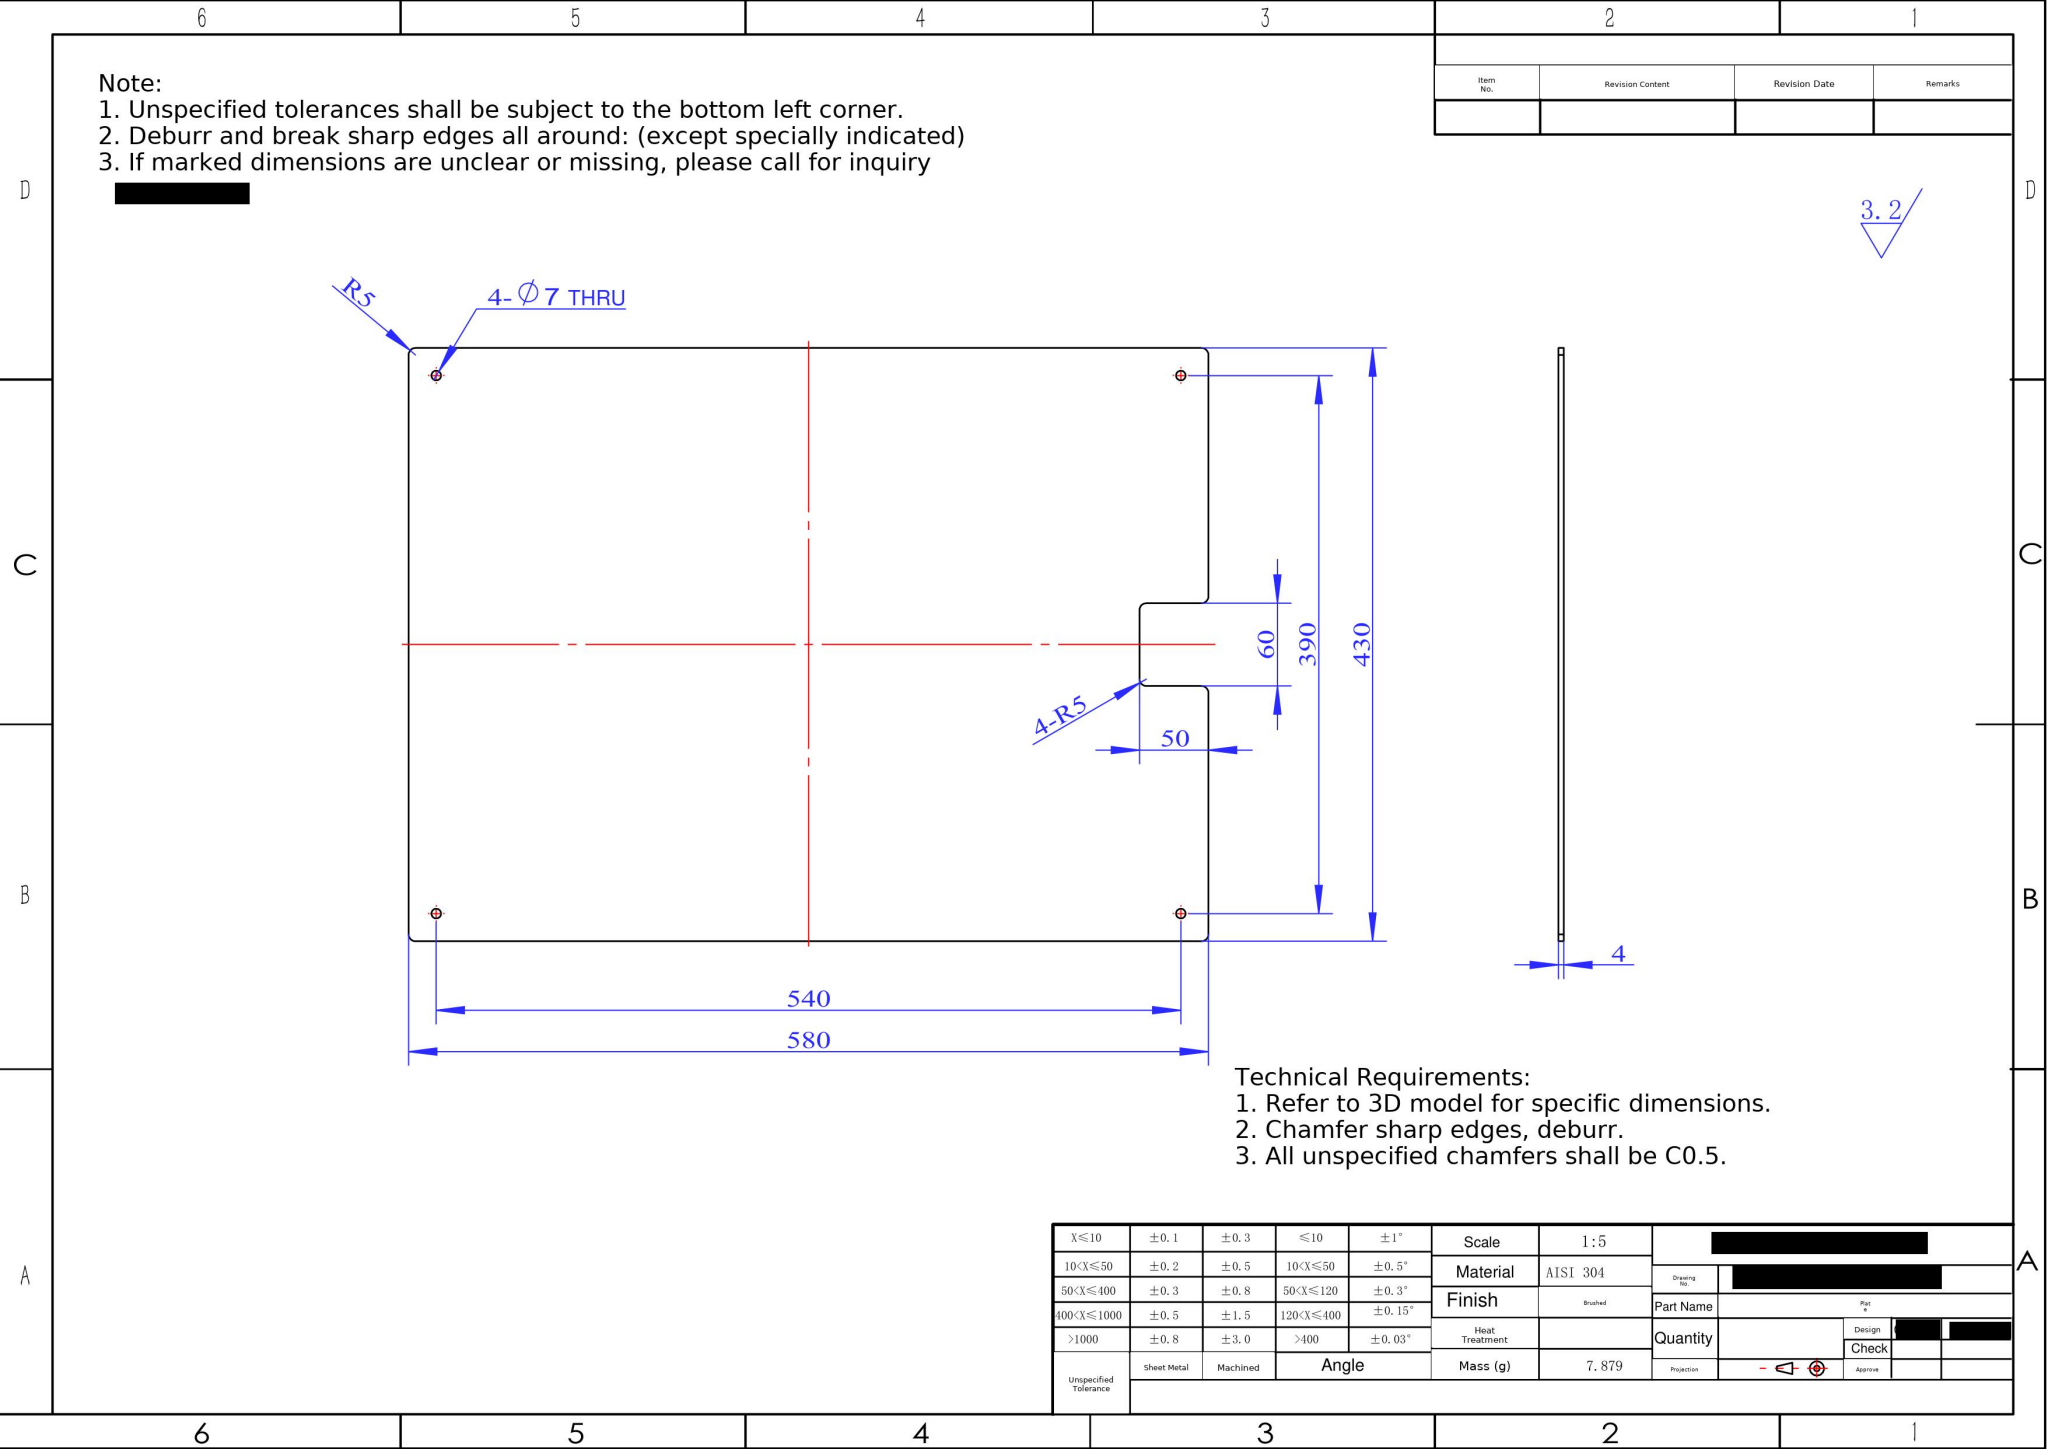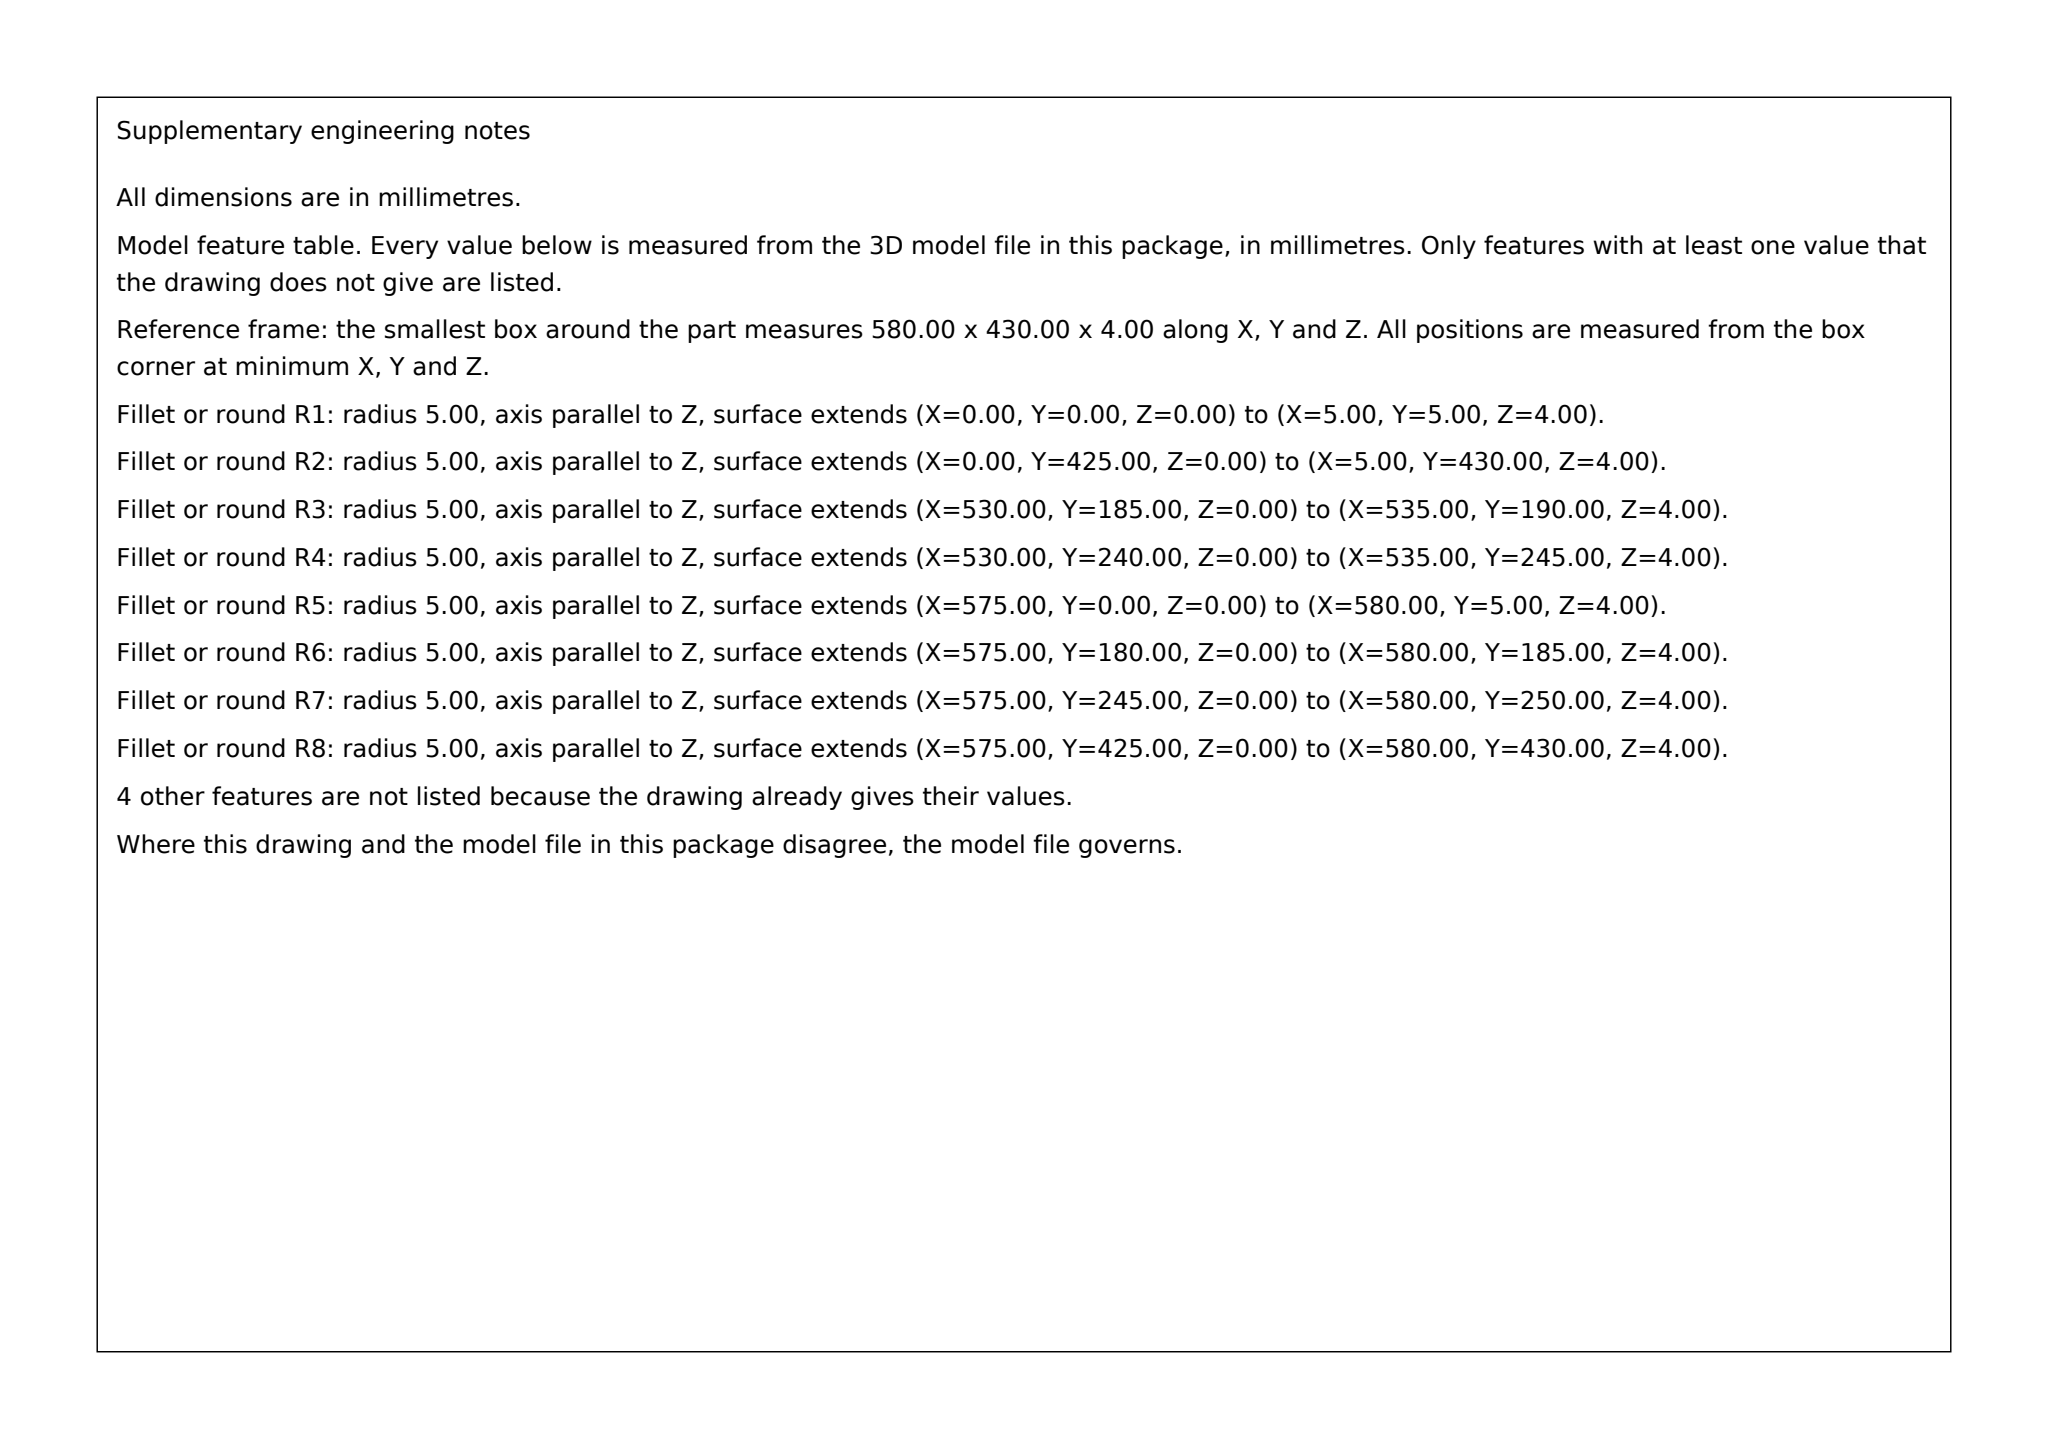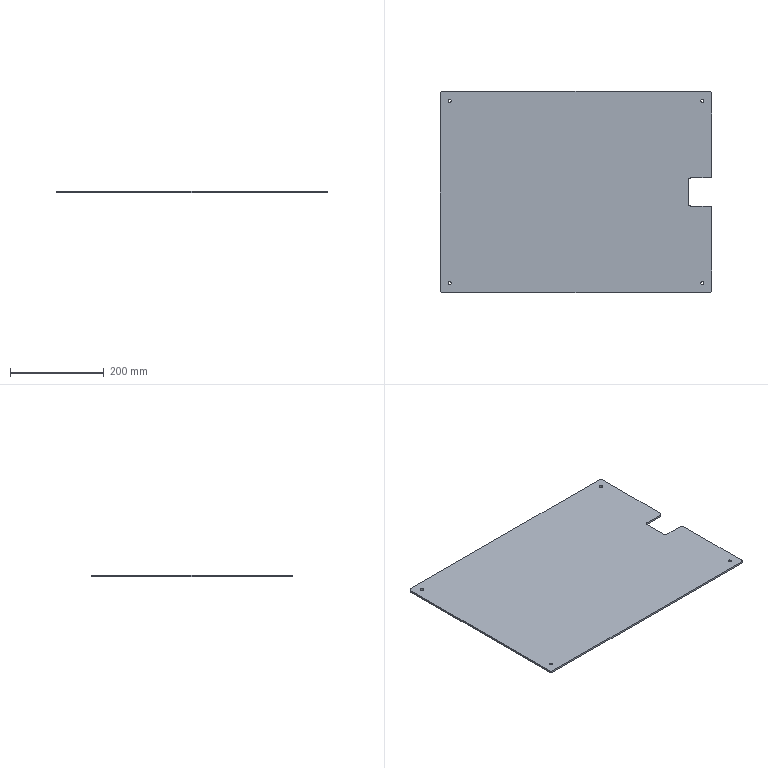Part | SolidWorks | mm | material AISI 304 | 1 solid | 26 faces | box 580 x 430 x 4 mm | volume 984898 mm3 | cylinder 16 | plane 10 | commonest cylinder face diameters 7 x8 10 x8
build123d program:
from build123d import *

# Parameters (mm, degrees)
SKETCH1_W           = 580
SKETCH1_H           = 430
BOSS_EXTRUDE1_DEPTH = 4
FILLET1_R           = 5
SKETCH2_W           = 50
SKETCH2_H           = 60
CUT_EXTRUDE1_DEPTH  = 723.022
FILLET2_R           = 5
SKETCH3_R           = 3.5
CUT_EXTRUDE2_DEPTH  = 723.022


with BuildPart() as part:
    # Sketch1 → Boss-Extrude1 (new body)
    with BuildSketch(Plane.XY):
        with Locations((290, -215)):
            Rectangle(SKETCH1_W, SKETCH1_H)
    extrude(amount=BOSS_EXTRUDE1_DEPTH)

    # Fillet1
    fillet1_edges = [part.edges().sort_by_distance(p)[0] for p in [
        (580, -430, 2),
        (0, -430, 2),
        (0, 0, 2),
        (580, 0, 2),
    ]]
    fillet(fillet1_edges, radius=FILLET1_R)

    # Sketch2 → Cut-Extrude1 (cut, through all)
    with BuildSketch(Plane(origin=(0, 0, 0), x_dir=(-1, 0, 0), z_dir=(0, 0, -1))):
        with Locations((-555, -215)):
            Rectangle(SKETCH2_W, SKETCH2_H)
    extrude(amount=-CUT_EXTRUDE1_DEPTH, mode=Mode.SUBTRACT)

    # Fillet2
    fillet2_edges = [part.edges().sort_by_distance(p)[0] for p in [
        (580, -245, 2),
        (580, -185, 2),
        (530, -185, 2),
        (530, -245, 2),
    ]]
    fillet(fillet2_edges, radius=FILLET2_R)

    # Sketch3 → Cut-Extrude2 (cut, through all)
    with BuildSketch(Plane(origin=(0, 0, 0), x_dir=(-1, 0, 0), z_dir=(0, 0, -1))):
        with Locations((-560, -20)):
            Circle(SKETCH3_R)
        with Locations((-560, -410)):
            Circle(SKETCH3_R)
        with Locations((-20, -20)):
            Circle(SKETCH3_R)
        with Locations((-20, -410)):
            Circle(SKETCH3_R)
    extrude(amount=-CUT_EXTRUDE2_DEPTH, mode=Mode.SUBTRACT)


solid = part.part
STEP:
#1=CARTESIAN_POINT('',(563.5,-410.,4.));
#2=VERTEX_POINT('',#1);
#3=CARTESIAN_POINT('',(556.5,-410.,4.));
#4=VERTEX_POINT('',#3);
#5=CARTESIAN_POINT('',(560.,-410.,4.));
#6=DIRECTION('',(0.,0.,-1.));
#7=DIRECTION('',(-1.,0.,0.));
#8=AXIS2_PLACEMENT_3D('',#5,#6,#7);
#9=CIRCLE('',#8,3.5);
#10=EDGE_CURVE('',#2,#4,#9,.T.);
#11=ORIENTED_EDGE('',*,*,#10,.F.);
#12=CARTESIAN_POINT('',(563.5,-410.,0.));
#13=VERTEX_POINT('',#12);
#14=CARTESIAN_POINT('',(563.5,-410.,4.));
#15=DIRECTION('',(0.,0.,-1.));
#16=VECTOR('',#15,1000.);
#17=LINE('',#14,#16);
#18=EDGE_CURVE('',#2,#13,#17,.T.);
#19=ORIENTED_EDGE('',*,*,#18,.T.);
#20=CARTESIAN_POINT('',(556.5,-410.,0.));
#21=VERTEX_POINT('',#20);
#22=CARTESIAN_POINT('',(560.,-410.,0.));
#23=DIRECTION('',(0.,0.,-1.));
#24=DIRECTION('',(-1.,0.,0.));
#25=AXIS2_PLACEMENT_3D('',#22,#23,#24);
#26=CIRCLE('',#25,3.5);
#27=EDGE_CURVE('',#13,#21,#26,.T.);
#28=ORIENTED_EDGE('',*,*,#27,.T.);
#29=CARTESIAN_POINT('',(556.5,-410.,4.));
#30=DIRECTION('',(0.,0.,-1.));
#31=VECTOR('',#30,1000.);
#32=LINE('',#29,#31);
#33=EDGE_CURVE('',#4,#21,#32,.T.);
#34=ORIENTED_EDGE('',*,*,#33,.F.);
#35=EDGE_LOOP('',(#11,#19,#28,#34));
#36=FACE_OUTER_BOUND('',#35,.T.);
#37=CARTESIAN_POINT('',(560.,-410.,4.));
#38=DIRECTION('',(0.,0.,-1.));
#39=DIRECTION('',(-1.,0.,0.));
#40=AXIS2_PLACEMENT_3D('',#37,#38,#39);
#41=CYLINDRICAL_SURFACE('',#40,3.5);
#42=ADVANCED_FACE('',(#36),#41,.F.);
#43=CARTESIAN_POINT('',(23.5,-20.,4.));
#44=VERTEX_POINT('',#43);
#45=CARTESIAN_POINT('',(16.5,-20.,4.));
#46=VERTEX_POINT('',#45);
#47=CARTESIAN_POINT('',(20.,-20.,4.));
#48=DIRECTION('',(0.,0.,-1.));
#49=DIRECTION('',(-1.,0.,0.));
#50=AXIS2_PLACEMENT_3D('',#47,#48,#49);
#51=CIRCLE('',#50,3.5);
#52=EDGE_CURVE('',#44,#46,#51,.T.);
#53=ORIENTED_EDGE('',*,*,#52,.F.);
#54=CARTESIAN_POINT('',(23.5,-20.,0.));
#55=VERTEX_POINT('',#54);
#56=CARTESIAN_POINT('',(23.5,-20.,4.));
#57=DIRECTION('',(0.,0.,-1.));
#58=VECTOR('',#57,1000.);
#59=LINE('',#56,#58);
#60=EDGE_CURVE('',#44,#55,#59,.T.);
#61=ORIENTED_EDGE('',*,*,#60,.T.);
#62=CARTESIAN_POINT('',(16.5,-20.,0.));
#63=VERTEX_POINT('',#62);
#64=CARTESIAN_POINT('',(20.,-20.,0.));
#65=DIRECTION('',(0.,0.,-1.));
#66=DIRECTION('',(-1.,0.,0.));
#67=AXIS2_PLACEMENT_3D('',#64,#65,#66);
#68=CIRCLE('',#67,3.5);
#69=EDGE_CURVE('',#55,#63,#68,.T.);
#70=ORIENTED_EDGE('',*,*,#69,.T.);
#71=CARTESIAN_POINT('',(16.5,-20.,4.));
#72=DIRECTION('',(0.,0.,-1.));
#73=VECTOR('',#72,1000.);
#74=LINE('',#71,#73);
#75=EDGE_CURVE('',#46,#63,#74,.T.);
#76=ORIENTED_EDGE('',*,*,#75,.F.);
#77=EDGE_LOOP('',(#53,#61,#70,#76));
#78=FACE_OUTER_BOUND('',#77,.T.);
#79=CARTESIAN_POINT('',(20.,-20.,4.));
#80=DIRECTION('',(0.,0.,-1.));
#81=DIRECTION('',(-1.,0.,0.));
#82=AXIS2_PLACEMENT_3D('',#79,#80,#81);
#83=CYLINDRICAL_SURFACE('',#82,3.5);
#84=ADVANCED_FACE('',(#78),#83,.F.);
#85=CARTESIAN_POINT('',(23.5,-410.,4.));
#86=VERTEX_POINT('',#85);
#87=CARTESIAN_POINT('',(16.5,-410.,4.));
#88=VERTEX_POINT('',#87);
#89=CARTESIAN_POINT('',(20.,-410.,4.));
#90=DIRECTION('',(0.,0.,-1.));
#91=DIRECTION('',(-1.,0.,0.));
#92=AXIS2_PLACEMENT_3D('',#89,#90,#91);
#93=CIRCLE('',#92,3.5);
#94=EDGE_CURVE('',#86,#88,#93,.T.);
#95=ORIENTED_EDGE('',*,*,#94,.F.);
#96=CARTESIAN_POINT('',(23.5,-410.,0.));
#97=VERTEX_POINT('',#96);
#98=CARTESIAN_POINT('',(23.5,-410.,4.));
#99=DIRECTION('',(0.,0.,-1.));
#100=VECTOR('',#99,1000.);
#101=LINE('',#98,#100);
#102=EDGE_CURVE('',#86,#97,#101,.T.);
#103=ORIENTED_EDGE('',*,*,#102,.T.);
#104=CARTESIAN_POINT('',(16.5,-410.,0.));
#105=VERTEX_POINT('',#104);
#106=CARTESIAN_POINT('',(20.,-410.,0.));
#107=DIRECTION('',(0.,0.,-1.));
#108=DIRECTION('',(-1.,0.,0.));
#109=AXIS2_PLACEMENT_3D('',#106,#107,#108);
#110=CIRCLE('',#109,3.5);
#111=EDGE_CURVE('',#97,#105,#110,.T.);
#112=ORIENTED_EDGE('',*,*,#111,.T.);
#113=CARTESIAN_POINT('',(16.5,-410.,4.));
#114=DIRECTION('',(0.,0.,-1.));
#115=VECTOR('',#114,1000.);
#116=LINE('',#113,#115);
#117=EDGE_CURVE('',#88,#105,#116,.T.);
#118=ORIENTED_EDGE('',*,*,#117,.F.);
#119=EDGE_LOOP('',(#95,#103,#112,#118));
#120=FACE_OUTER_BOUND('',#119,.T.);
#121=CARTESIAN_POINT('',(20.,-410.,4.));
#122=DIRECTION('',(0.,0.,-1.));
#123=DIRECTION('',(-1.,0.,0.));
#124=AXIS2_PLACEMENT_3D('',#121,#122,#123);
#125=CYLINDRICAL_SURFACE('',#124,3.5);
#126=ADVANCED_FACE('',(#120),#125,.F.);
#127=CARTESIAN_POINT('',(563.5,-20.,4.));
#128=VERTEX_POINT('',#127);
#129=CARTESIAN_POINT('',(556.5,-20.,4.));
#130=VERTEX_POINT('',#129);
#131=CARTESIAN_POINT('',(560.,-20.,4.));
#132=DIRECTION('',(0.,0.,-1.));
#133=DIRECTION('',(-1.,0.,0.));
#134=AXIS2_PLACEMENT_3D('',#131,#132,#133);
#135=CIRCLE('',#134,3.5);
#136=EDGE_CURVE('',#128,#130,#135,.T.);
#137=ORIENTED_EDGE('',*,*,#136,.F.);
#138=CARTESIAN_POINT('',(563.5,-20.,0.));
#139=VERTEX_POINT('',#138);
#140=CARTESIAN_POINT('',(563.5,-20.,4.));
#141=DIRECTION('',(0.,0.,-1.));
#142=VECTOR('',#141,1000.);
#143=LINE('',#140,#142);
#144=EDGE_CURVE('',#128,#139,#143,.T.);
#145=ORIENTED_EDGE('',*,*,#144,.T.);
#146=CARTESIAN_POINT('',(556.5,-20.,0.));
#147=VERTEX_POINT('',#146);
#148=CARTESIAN_POINT('',(560.,-20.,0.));
#149=DIRECTION('',(0.,0.,-1.));
#150=DIRECTION('',(-1.,0.,0.));
#151=AXIS2_PLACEMENT_3D('',#148,#149,#150);
#152=CIRCLE('',#151,3.5);
#153=EDGE_CURVE('',#139,#147,#152,.T.);
#154=ORIENTED_EDGE('',*,*,#153,.T.);
#155=CARTESIAN_POINT('',(556.5,-20.,4.));
#156=DIRECTION('',(0.,0.,-1.));
#157=VECTOR('',#156,1000.);
#158=LINE('',#155,#157);
#159=EDGE_CURVE('',#130,#147,#158,.T.);
#160=ORIENTED_EDGE('',*,*,#159,.F.);
#161=EDGE_LOOP('',(#137,#145,#154,#160));
#162=FACE_OUTER_BOUND('',#161,.T.);
#163=CARTESIAN_POINT('',(560.,-20.,4.));
#164=DIRECTION('',(0.,0.,-1.));
#165=DIRECTION('',(-1.,0.,0.));
#166=AXIS2_PLACEMENT_3D('',#163,#164,#165);
#167=CYLINDRICAL_SURFACE('',#166,3.5);
#168=ADVANCED_FACE('',(#162),#167,.F.);
#169=CARTESIAN_POINT('',(580.,-180.,4.));
#170=VERTEX_POINT('',#169);
#171=CARTESIAN_POINT('',(580.,-5.,4.));
#172=VERTEX_POINT('',#171);
#173=CARTESIAN_POINT('',(580.,-430.,4.));
#174=DIRECTION('',(0.,1.,0.));
#175=VECTOR('',#174,1000.);
#176=LINE('',#173,#175);
#177=EDGE_CURVE('',#170,#172,#176,.T.);
#178=ORIENTED_EDGE('',*,*,#177,.F.);
#179=CARTESIAN_POINT('',(580.,-180.,0.));
#180=VERTEX_POINT('',#179);
#181=CARTESIAN_POINT('',(580.,-180.,4.));
#182=DIRECTION('',(0.,0.,-1.));
#183=VECTOR('',#182,1000.);
#184=LINE('',#181,#183);
#185=EDGE_CURVE('',#170,#180,#184,.T.);
#186=ORIENTED_EDGE('',*,*,#185,.T.);
#187=CARTESIAN_POINT('',(580.,-5.,0.));
#188=VERTEX_POINT('',#187);
#189=CARTESIAN_POINT('',(580.,-430.,0.));
#190=DIRECTION('',(0.,1.,0.));
#191=VECTOR('',#190,1000.);
#192=LINE('',#189,#191);
#193=EDGE_CURVE('',#180,#188,#192,.T.);
#194=ORIENTED_EDGE('',*,*,#193,.T.);
#195=CARTESIAN_POINT('',(580.,-5.,4.));
#196=DIRECTION('',(0.,0.,1.));
#197=VECTOR('',#196,1000.);
#198=LINE('',#195,#197);
#199=EDGE_CURVE('',#188,#172,#198,.T.);
#200=ORIENTED_EDGE('',*,*,#199,.T.);
#201=EDGE_LOOP('',(#178,#186,#194,#200));
#202=FACE_OUTER_BOUND('',#201,.T.);
#203=CARTESIAN_POINT('',(580.,-430.,4.));
#204=DIRECTION('',(-1.,0.,0.));
#205=DIRECTION('',(0.,0.,1.));
#206=AXIS2_PLACEMENT_3D('',#203,#204,#205);
#207=PLANE('',#206);
#208=ADVANCED_FACE('',(#202),#207,.F.);
#209=CARTESIAN_POINT('',(580.,-425.,0.));
#210=VERTEX_POINT('',#209);
#211=CARTESIAN_POINT('',(580.,-250.,0.));
#212=VERTEX_POINT('',#211);
#213=CARTESIAN_POINT('',(580.,-430.,0.));
#214=DIRECTION('',(0.,1.,0.));
#215=VECTOR('',#214,1000.);
#216=LINE('',#213,#215);
#217=EDGE_CURVE('',#210,#212,#216,.T.);
#218=ORIENTED_EDGE('',*,*,#217,.T.);
#219=CARTESIAN_POINT('',(580.,-250.,4.));
#220=VERTEX_POINT('',#219);
#221=CARTESIAN_POINT('',(580.,-250.,4.));
#222=DIRECTION('',(0.,0.,1.));
#223=VECTOR('',#222,1000.);
#224=LINE('',#221,#223);
#225=EDGE_CURVE('',#212,#220,#224,.T.);
#226=ORIENTED_EDGE('',*,*,#225,.T.);
#227=CARTESIAN_POINT('',(580.,-425.,4.));
#228=VERTEX_POINT('',#227);
#229=CARTESIAN_POINT('',(580.,-430.,4.));
#230=DIRECTION('',(0.,1.,0.));
#231=VECTOR('',#230,1000.);
#232=LINE('',#229,#231);
#233=EDGE_CURVE('',#228,#220,#232,.T.);
#234=ORIENTED_EDGE('',*,*,#233,.F.);
#235=CARTESIAN_POINT('',(580.,-425.,4.));
#236=DIRECTION('',(0.,0.,-1.));
#237=VECTOR('',#236,1000.);
#238=LINE('',#235,#237);
#239=EDGE_CURVE('',#228,#210,#238,.T.);
#240=ORIENTED_EDGE('',*,*,#239,.T.);
#241=EDGE_LOOP('',(#218,#226,#234,#240));
#242=FACE_OUTER_BOUND('',#241,.T.);
#243=CARTESIAN_POINT('',(580.,-430.,4.));
#244=DIRECTION('',(-1.,0.,0.));
#245=DIRECTION('',(0.,0.,1.));
#246=AXIS2_PLACEMENT_3D('',#243,#244,#245);
#247=PLANE('',#246);
#248=ADVANCED_FACE('',(#242),#247,.F.);
#249=CARTESIAN_POINT('',(575.,0.,4.));
#250=VERTEX_POINT('',#249);
#251=CARTESIAN_POINT('',(5.,0.,4.));
#252=VERTEX_POINT('',#251);
#253=CARTESIAN_POINT('',(580.,0.,4.));
#254=DIRECTION('',(-1.,-0.,0.));
#255=VECTOR('',#254,1000.);
#256=LINE('',#253,#255);
#257=EDGE_CURVE('',#250,#252,#256,.T.);
#258=ORIENTED_EDGE('',*,*,#257,.F.);
#259=CARTESIAN_POINT('',(575.,0.,0.));
#260=VERTEX_POINT('',#259);
#261=CARTESIAN_POINT('',(575.,0.,4.));
#262=DIRECTION('',(0.,0.,-1.));
#263=VECTOR('',#262,1000.);
#264=LINE('',#261,#263);
#265=EDGE_CURVE('',#250,#260,#264,.T.);
#266=ORIENTED_EDGE('',*,*,#265,.T.);
#267=CARTESIAN_POINT('',(5.,0.,0.));
#268=VERTEX_POINT('',#267);
#269=CARTESIAN_POINT('',(580.,0.,0.));
#270=DIRECTION('',(-1.,-0.,0.));
#271=VECTOR('',#270,1000.);
#272=LINE('',#269,#271);
#273=EDGE_CURVE('',#260,#268,#272,.T.);
#274=ORIENTED_EDGE('',*,*,#273,.T.);
#275=CARTESIAN_POINT('',(5.,0.,4.));
#276=DIRECTION('',(0.,0.,1.));
#277=VECTOR('',#276,1000.);
#278=LINE('',#275,#277);
#279=EDGE_CURVE('',#268,#252,#278,.T.);
#280=ORIENTED_EDGE('',*,*,#279,.T.);
#281=EDGE_LOOP('',(#258,#266,#274,#280));
#282=FACE_OUTER_BOUND('',#281,.T.);
#283=CARTESIAN_POINT('',(580.,0.,4.));
#284=DIRECTION('',(0.,-1.,0.));
#285=DIRECTION('',(1.,0.,0.));
#286=AXIS2_PLACEMENT_3D('',#283,#284,#285);
#287=PLANE('',#286);
#288=ADVANCED_FACE('',(#282),#287,.F.);
#289=CARTESIAN_POINT('',(0.,-5.,0.));
#290=VERTEX_POINT('',#289);
#291=CARTESIAN_POINT('',(0.,-425.,0.));
#292=VERTEX_POINT('',#291);
#293=CARTESIAN_POINT('',(0.,-430.,0.));
#294=DIRECTION('',(0.,-1.,0.));
#295=VECTOR('',#294,1000.);
#296=LINE('',#293,#295);
#297=EDGE_CURVE('',#290,#292,#296,.T.);
#298=ORIENTED_EDGE('',*,*,#297,.T.);
#299=CARTESIAN_POINT('',(0.,-425.,4.));
#300=VERTEX_POINT('',#299);
#301=CARTESIAN_POINT('',(0.,-425.,4.));
#302=DIRECTION('',(0.,0.,1.));
#303=VECTOR('',#302,1000.);
#304=LINE('',#301,#303);
#305=EDGE_CURVE('',#292,#300,#304,.T.);
#306=ORIENTED_EDGE('',*,*,#305,.T.);
#307=CARTESIAN_POINT('',(0.,-5.,4.));
#308=VERTEX_POINT('',#307);
#309=CARTESIAN_POINT('',(0.,-430.,4.));
#310=DIRECTION('',(0.,-1.,0.));
#311=VECTOR('',#310,1000.);
#312=LINE('',#309,#311);
#313=EDGE_CURVE('',#308,#300,#312,.T.);
#314=ORIENTED_EDGE('',*,*,#313,.F.);
#315=CARTESIAN_POINT('',(0.,-5.,4.));
#316=DIRECTION('',(0.,0.,-1.));
#317=VECTOR('',#316,1000.);
#318=LINE('',#315,#317);
#319=EDGE_CURVE('',#308,#290,#318,.T.);
#320=ORIENTED_EDGE('',*,*,#319,.T.);
#321=EDGE_LOOP('',(#298,#306,#314,#320));
#322=FACE_OUTER_BOUND('',#321,.T.);
#323=CARTESIAN_POINT('',(0.,-430.,4.));
#324=DIRECTION('',(1.,0.,0.));
#325=DIRECTION('',(0.,0.,-1.));
#326=AXIS2_PLACEMENT_3D('',#323,#324,#325);
#327=PLANE('',#326);
#328=ADVANCED_FACE('',(#322),#327,.F.);
#329=CARTESIAN_POINT('',(5.,-430.,4.));
#330=VERTEX_POINT('',#329);
#331=CARTESIAN_POINT('',(575.,-430.,4.));
#332=VERTEX_POINT('',#331);
#333=CARTESIAN_POINT('',(580.,-430.,4.));
#334=DIRECTION('',(1.,0.,0.));
#335=VECTOR('',#334,1000.);
#336=LINE('',#333,#335);
#337=EDGE_CURVE('',#330,#332,#336,.T.);
#338=ORIENTED_EDGE('',*,*,#337,.F.);
#339=CARTESIAN_POINT('',(5.,-430.,0.));
#340=VERTEX_POINT('',#339);
#341=CARTESIAN_POINT('',(5.,-430.,4.));
#342=DIRECTION('',(0.,0.,-1.));
#343=VECTOR('',#342,1000.);
#344=LINE('',#341,#343);
#345=EDGE_CURVE('',#330,#340,#344,.T.);
#346=ORIENTED_EDGE('',*,*,#345,.T.);
#347=CARTESIAN_POINT('',(575.,-430.,0.));
#348=VERTEX_POINT('',#347);
#349=CARTESIAN_POINT('',(580.,-430.,0.));
#350=DIRECTION('',(1.,0.,0.));
#351=VECTOR('',#350,1000.);
#352=LINE('',#349,#351);
#353=EDGE_CURVE('',#340,#348,#352,.T.);
#354=ORIENTED_EDGE('',*,*,#353,.T.);
#355=CARTESIAN_POINT('',(575.,-430.,4.));
#356=DIRECTION('',(0.,0.,1.));
#357=VECTOR('',#356,1000.);
#358=LINE('',#355,#357);
#359=EDGE_CURVE('',#348,#332,#358,.T.);
#360=ORIENTED_EDGE('',*,*,#359,.T.);
#361=EDGE_LOOP('',(#338,#346,#354,#360));
#362=FACE_OUTER_BOUND('',#361,.T.);
#363=CARTESIAN_POINT('',(580.,-430.,4.));
#364=DIRECTION('',(-0.,1.,0.));
#365=DIRECTION('',(-1.,-0.,0.));
#366=AXIS2_PLACEMENT_3D('',#363,#364,#365);
#367=PLANE('',#366);
#368=ADVANCED_FACE('',(#362),#367,.F.);
#369=CARTESIAN_POINT('',(560.,-410.,4.));
#370=DIRECTION('',(0.,0.,-1.));
#371=DIRECTION('',(-1.,0.,0.));
#372=AXIS2_PLACEMENT_3D('',#369,#370,#371);
#373=CIRCLE('',#372,3.5);
#374=EDGE_CURVE('',#4,#2,#373,.T.);
#375=ORIENTED_EDGE('',*,*,#374,.T.);
#376=ORIENTED_EDGE('',*,*,#10,.T.);
#377=EDGE_LOOP('',(#375,#376));
#378=FACE_BOUND('',#377,.T.);
#379=CARTESIAN_POINT('',(20.,-20.,4.));
#380=DIRECTION('',(0.,0.,-1.));
#381=DIRECTION('',(-1.,0.,0.));
#382=AXIS2_PLACEMENT_3D('',#379,#380,#381);
#383=CIRCLE('',#382,3.5);
#384=EDGE_CURVE('',#46,#44,#383,.T.);
#385=ORIENTED_EDGE('',*,*,#384,.T.);
#386=ORIENTED_EDGE('',*,*,#52,.T.);
#387=EDGE_LOOP('',(#385,#386));
#388=FACE_BOUND('',#387,.T.);
#389=CARTESIAN_POINT('',(20.,-410.,4.));
#390=DIRECTION('',(0.,0.,-1.));
#391=DIRECTION('',(-1.,0.,0.));
#392=AXIS2_PLACEMENT_3D('',#389,#390,#391);
#393=CIRCLE('',#392,3.5);
#394=EDGE_CURVE('',#88,#86,#393,.T.);
#395=ORIENTED_EDGE('',*,*,#394,.T.);
#396=ORIENTED_EDGE('',*,*,#94,.T.);
#397=EDGE_LOOP('',(#395,#396));
#398=FACE_BOUND('',#397,.T.);
#399=CARTESIAN_POINT('',(560.,-20.,4.));
#400=DIRECTION('',(0.,0.,-1.));
#401=DIRECTION('',(-1.,0.,0.));
#402=AXIS2_PLACEMENT_3D('',#399,#400,#401);
#403=CIRCLE('',#402,3.5);
#404=EDGE_CURVE('',#130,#128,#403,.T.);
#405=ORIENTED_EDGE('',*,*,#404,.T.);
#406=ORIENTED_EDGE('',*,*,#136,.T.);
#407=EDGE_LOOP('',(#405,#406));
#408=FACE_BOUND('',#407,.T.);
#409=ORIENTED_EDGE('',*,*,#233,.T.);
#410=CARTESIAN_POINT('',(575.,-245.,4.));
#411=VERTEX_POINT('',#410);
#412=CARTESIAN_POINT('',(575.,-250.,4.));
#413=DIRECTION('',(0.,0.,1.));
#414=DIRECTION('',(1.,0.,0.));
#415=AXIS2_PLACEMENT_3D('',#412,#413,#414);
#416=CIRCLE('',#415,5.);
#417=EDGE_CURVE('',#220,#411,#416,.T.);
#418=ORIENTED_EDGE('',*,*,#417,.T.);
#419=CARTESIAN_POINT('',(535.,-245.,4.));
#420=VERTEX_POINT('',#419);
#421=CARTESIAN_POINT('',(580.,-245.,4.));
#422=DIRECTION('',(-1.,0.,0.));
#423=VECTOR('',#422,1000.);
#424=LINE('',#421,#423);
#425=EDGE_CURVE('',#411,#420,#424,.T.);
#426=ORIENTED_EDGE('',*,*,#425,.T.);
#427=CARTESIAN_POINT('',(530.,-240.,4.));
#428=VERTEX_POINT('',#427);
#429=CARTESIAN_POINT('',(535.,-240.,4.));
#430=DIRECTION('',(0.,0.,-1.));
#431=DIRECTION('',(1.,0.,0.));
#432=AXIS2_PLACEMENT_3D('',#429,#430,#431);
#433=CIRCLE('',#432,5.);
#434=EDGE_CURVE('',#420,#428,#433,.T.);
#435=ORIENTED_EDGE('',*,*,#434,.T.);
#436=CARTESIAN_POINT('',(530.,-190.,4.));
#437=VERTEX_POINT('',#436);
#438=CARTESIAN_POINT('',(530.,-185.,4.));
#439=DIRECTION('',(0.,1.,0.));
#440=VECTOR('',#439,1000.);
#441=LINE('',#438,#440);
#442=EDGE_CURVE('',#428,#437,#441,.T.);
#443=ORIENTED_EDGE('',*,*,#442,.T.);
#444=CARTESIAN_POINT('',(535.,-185.,4.));
#445=VERTEX_POINT('',#444);
#446=CARTESIAN_POINT('',(535.,-190.,4.));
#447=DIRECTION('',(0.,0.,-1.));
#448=DIRECTION('',(1.,0.,0.));
#449=AXIS2_PLACEMENT_3D('',#446,#447,#448);
#450=CIRCLE('',#449,5.);
#451=EDGE_CURVE('',#437,#445,#450,.T.);
#452=ORIENTED_EDGE('',*,*,#451,.T.);
#453=CARTESIAN_POINT('',(575.,-185.,4.));
#454=VERTEX_POINT('',#453);
#455=CARTESIAN_POINT('',(580.,-185.,4.));
#456=DIRECTION('',(1.,-0.,0.));
#457=VECTOR('',#456,1000.);
#458=LINE('',#455,#457);
#459=EDGE_CURVE('',#445,#454,#458,.T.);
#460=ORIENTED_EDGE('',*,*,#459,.T.);
#461=CARTESIAN_POINT('',(575.,-180.,4.));
#462=DIRECTION('',(0.,0.,1.));
#463=DIRECTION('',(1.,0.,0.));
#464=AXIS2_PLACEMENT_3D('',#461,#462,#463);
#465=CIRCLE('',#464,5.);
#466=EDGE_CURVE('',#454,#170,#465,.T.);
#467=ORIENTED_EDGE('',*,*,#466,.T.);
#468=ORIENTED_EDGE('',*,*,#177,.T.);
#469=CARTESIAN_POINT('',(575.,-5.,4.));
#470=DIRECTION('',(0.,0.,1.));
#471=DIRECTION('',(1.,0.,0.));
#472=AXIS2_PLACEMENT_3D('',#469,#470,#471);
#473=CIRCLE('',#472,5.);
#474=EDGE_CURVE('',#172,#250,#473,.T.);
#475=ORIENTED_EDGE('',*,*,#474,.T.);
#476=ORIENTED_EDGE('',*,*,#257,.T.);
#477=CARTESIAN_POINT('',(5.,-5.,4.));
#478=DIRECTION('',(0.,0.,1.));
#479=DIRECTION('',(1.,0.,0.));
#480=AXIS2_PLACEMENT_3D('',#477,#478,#479);
#481=CIRCLE('',#480,5.);
#482=EDGE_CURVE('',#252,#308,#481,.T.);
#483=ORIENTED_EDGE('',*,*,#482,.T.);
#484=ORIENTED_EDGE('',*,*,#313,.T.);
#485=CARTESIAN_POINT('',(5.,-425.,4.));
#486=DIRECTION('',(0.,0.,1.));
#487=DIRECTION('',(1.,0.,0.));
#488=AXIS2_PLACEMENT_3D('',#485,#486,#487);
#489=CIRCLE('',#488,5.);
#490=EDGE_CURVE('',#300,#330,#489,.T.);
#491=ORIENTED_EDGE('',*,*,#490,.T.);
#492=ORIENTED_EDGE('',*,*,#337,.T.);
#493=CARTESIAN_POINT('',(575.,-425.,4.));
#494=DIRECTION('',(0.,0.,1.));
#495=DIRECTION('',(1.,0.,0.));
#496=AXIS2_PLACEMENT_3D('',#493,#494,#495);
#497=CIRCLE('',#496,5.);
#498=EDGE_CURVE('',#332,#228,#497,.T.);
#499=ORIENTED_EDGE('',*,*,#498,.T.);
#500=EDGE_LOOP('',(#409,#418,#426,#435,#443,#452,#460,#467,#468,#475,#476,#483,#484,#491,#492,#499));
#501=FACE_OUTER_BOUND('',#500,.T.);
#502=CARTESIAN_POINT('',(0.,0.,4.));
#503=DIRECTION('',(0.,0.,1.));
#504=DIRECTION('',(1.,0.,0.));
#505=AXIS2_PLACEMENT_3D('',#502,#503,#504);
#506=PLANE('',#505);
#507=ADVANCED_FACE('',(#378,#388,#398,#408,#501),#506,.T.);
#508=CARTESIAN_POINT('',(560.,-410.,0.));
#509=DIRECTION('',(0.,0.,-1.));
#510=DIRECTION('',(-1.,0.,0.));
#511=AXIS2_PLACEMENT_3D('',#508,#509,#510);
#512=CIRCLE('',#511,3.5);
#513=EDGE_CURVE('',#21,#13,#512,.T.);
#514=ORIENTED_EDGE('',*,*,#513,.F.);
#515=ORIENTED_EDGE('',*,*,#27,.F.);
#516=EDGE_LOOP('',(#514,#515));
#517=FACE_BOUND('',#516,.T.);
#518=CARTESIAN_POINT('',(20.,-20.,0.));
#519=DIRECTION('',(0.,0.,-1.));
#520=DIRECTION('',(-1.,0.,0.));
#521=AXIS2_PLACEMENT_3D('',#518,#519,#520);
#522=CIRCLE('',#521,3.5);
#523=EDGE_CURVE('',#63,#55,#522,.T.);
#524=ORIENTED_EDGE('',*,*,#523,.F.);
#525=ORIENTED_EDGE('',*,*,#69,.F.);
#526=EDGE_LOOP('',(#524,#525));
#527=FACE_BOUND('',#526,.T.);
#528=CARTESIAN_POINT('',(20.,-410.,0.));
#529=DIRECTION('',(0.,0.,-1.));
#530=DIRECTION('',(-1.,0.,0.));
#531=AXIS2_PLACEMENT_3D('',#528,#529,#530);
#532=CIRCLE('',#531,3.5);
#533=EDGE_CURVE('',#105,#97,#532,.T.);
#534=ORIENTED_EDGE('',*,*,#533,.F.);
#535=ORIENTED_EDGE('',*,*,#111,.F.);
#536=EDGE_LOOP('',(#534,#535));
#537=FACE_BOUND('',#536,.T.);
#538=CARTESIAN_POINT('',(560.,-20.,0.));
#539=DIRECTION('',(0.,0.,-1.));
#540=DIRECTION('',(-1.,0.,0.));
#541=AXIS2_PLACEMENT_3D('',#538,#539,#540);
#542=CIRCLE('',#541,3.5);
#543=EDGE_CURVE('',#147,#139,#542,.T.);
#544=ORIENTED_EDGE('',*,*,#543,.F.);
#545=ORIENTED_EDGE('',*,*,#153,.F.);
#546=EDGE_LOOP('',(#544,#545));
#547=FACE_BOUND('',#546,.T.);
#548=CARTESIAN_POINT('',(575.,-245.,0.));
#549=VERTEX_POINT('',#548);
#550=CARTESIAN_POINT('',(535.,-245.,0.));
#551=VERTEX_POINT('',#550);
#552=CARTESIAN_POINT('',(580.,-245.,0.));
#553=DIRECTION('',(-1.,0.,0.));
#554=VECTOR('',#553,1000.);
#555=LINE('',#552,#554);
#556=EDGE_CURVE('',#549,#551,#555,.T.);
#557=ORIENTED_EDGE('',*,*,#556,.F.);
#558=CARTESIAN_POINT('',(575.,-250.,0.));
#559=DIRECTION('',(0.,0.,-1.));
#560=DIRECTION('',(1.,0.,0.));
#561=AXIS2_PLACEMENT_3D('',#558,#559,#560);
#562=CIRCLE('',#561,5.);
#563=EDGE_CURVE('',#549,#212,#562,.T.);
#564=ORIENTED_EDGE('',*,*,#563,.T.);
#565=ORIENTED_EDGE('',*,*,#217,.F.);
#566=CARTESIAN_POINT('',(575.,-425.,0.));
#567=DIRECTION('',(0.,0.,-1.));
#568=DIRECTION('',(1.,0.,0.));
#569=AXIS2_PLACEMENT_3D('',#566,#567,#568);
#570=CIRCLE('',#569,5.);
#571=EDGE_CURVE('',#210,#348,#570,.T.);
#572=ORIENTED_EDGE('',*,*,#571,.T.);
#573=ORIENTED_EDGE('',*,*,#353,.F.);
#574=CARTESIAN_POINT('',(5.,-425.,0.));
#575=DIRECTION('',(0.,0.,-1.));
#576=DIRECTION('',(1.,0.,0.));
#577=AXIS2_PLACEMENT_3D('',#574,#575,#576);
#578=CIRCLE('',#577,5.);
#579=EDGE_CURVE('',#340,#292,#578,.T.);
#580=ORIENTED_EDGE('',*,*,#579,.T.);
#581=ORIENTED_EDGE('',*,*,#297,.F.);
#582=CARTESIAN_POINT('',(5.,-5.,0.));
#583=DIRECTION('',(0.,0.,-1.));
#584=DIRECTION('',(1.,0.,0.));
#585=AXIS2_PLACEMENT_3D('',#582,#583,#584);
#586=CIRCLE('',#585,5.);
#587=EDGE_CURVE('',#290,#268,#586,.T.);
#588=ORIENTED_EDGE('',*,*,#587,.T.);
#589=ORIENTED_EDGE('',*,*,#273,.F.);
#590=CARTESIAN_POINT('',(575.,-5.,0.));
#591=DIRECTION('',(0.,0.,-1.));
#592=DIRECTION('',(1.,0.,0.));
#593=AXIS2_PLACEMENT_3D('',#590,#591,#592);
#594=CIRCLE('',#593,5.);
#595=EDGE_CURVE('',#260,#188,#594,.T.);
#596=ORIENTED_EDGE('',*,*,#595,.T.);
#597=ORIENTED_EDGE('',*,*,#193,.F.);
#598=CARTESIAN_POINT('',(575.,-185.,0.));
#599=VERTEX_POINT('',#598);
#600=CARTESIAN_POINT('',(575.,-180.,0.));
#601=DIRECTION('',(0.,0.,-1.));
#602=DIRECTION('',(1.,-0.,0.));
#603=AXIS2_PLACEMENT_3D('',#600,#601,#602);
#604=CIRCLE('',#603,5.);
#605=EDGE_CURVE('',#180,#599,#604,.T.);
#606=ORIENTED_EDGE('',*,*,#605,.T.);
#607=CARTESIAN_POINT('',(535.,-185.,0.));
#608=VERTEX_POINT('',#607);
#609=CARTESIAN_POINT('',(580.,-185.,0.));
#610=DIRECTION('',(1.,-0.,0.));
#611=VECTOR('',#610,1000.);
#612=LINE('',#609,#611);
#613=EDGE_CURVE('',#608,#599,#612,.T.);
#614=ORIENTED_EDGE('',*,*,#613,.F.);
#615=CARTESIAN_POINT('',(530.,-190.,0.));
#616=VERTEX_POINT('',#615);
#617=CARTESIAN_POINT('',(535.,-190.,0.));
#618=DIRECTION('',(0.,0.,1.));
#619=DIRECTION('',(1.,0.,0.));
#620=AXIS2_PLACEMENT_3D('',#617,#618,#619);
#621=CIRCLE('',#620,5.);
#622=EDGE_CURVE('',#608,#616,#621,.T.);
#623=ORIENTED_EDGE('',*,*,#622,.T.);
#624=CARTESIAN_POINT('',(530.,-240.,0.));
#625=VERTEX_POINT('',#624);
#626=CARTESIAN_POINT('',(530.,-185.,0.));
#627=DIRECTION('',(0.,1.,0.));
#628=VECTOR('',#627,1000.);
#629=LINE('',#626,#628);
#630=EDGE_CURVE('',#625,#616,#629,.T.);
#631=ORIENTED_EDGE('',*,*,#630,.F.);
#632=CARTESIAN_POINT('',(535.,-240.,0.));
#633=DIRECTION('',(0.,0.,1.));
#634=DIRECTION('',(1.,0.,0.));
#635=AXIS2_PLACEMENT_3D('',#632,#633,#634);
#636=CIRCLE('',#635,5.);
#637=EDGE_CURVE('',#625,#551,#636,.T.);
#638=ORIENTED_EDGE('',*,*,#637,.T.);
#639=EDGE_LOOP('',(#557,#564,#565,#572,#573,#580,#581,#588,#589,#596,#597,#606,#614,#623,#631,#638));
#640=FACE_OUTER_BOUND('',#639,.T.);
#641=CARTESIAN_POINT('',(0.,0.,0.));
#642=DIRECTION('',(0.,0.,1.));
#643=DIRECTION('',(1.,0.,0.));
#644=AXIS2_PLACEMENT_3D('',#641,#642,#643);
#645=PLANE('',#644);
#646=ADVANCED_FACE('',(#517,#527,#537,#547,#640),#645,.F.);
#647=ORIENTED_EDGE('',*,*,#490,.F.);
#648=ORIENTED_EDGE('',*,*,#305,.F.);
#649=ORIENTED_EDGE('',*,*,#579,.F.);
#650=ORIENTED_EDGE('',*,*,#345,.F.);
#651=EDGE_LOOP('',(#647,#648,#649,#650));
#652=FACE_OUTER_BOUND('',#651,.T.);
#653=CARTESIAN_POINT('',(5.,-425.,4.));
#654=DIRECTION('',(0.,0.,-1.));
#655=DIRECTION('',(-1.,0.,0.));
#656=AXIS2_PLACEMENT_3D('',#653,#654,#655);
#657=CYLINDRICAL_SURFACE('',#656,5.);
#658=ADVANCED_FACE('',(#652),#657,.T.);
#659=ORIENTED_EDGE('',*,*,#498,.F.);
#660=ORIENTED_EDGE('',*,*,#359,.F.);
#661=ORIENTED_EDGE('',*,*,#571,.F.);
#662=ORIENTED_EDGE('',*,*,#239,.F.);
#663=EDGE_LOOP('',(#659,#660,#661,#662));
#664=FACE_OUTER_BOUND('',#663,.T.);
#665=CARTESIAN_POINT('',(575.,-425.,4.));
#666=DIRECTION('',(0.,0.,-1.));
#667=DIRECTION('',(-1.,0.,0.));
#668=AXIS2_PLACEMENT_3D('',#665,#666,#667);
#669=CYLINDRICAL_SURFACE('',#668,5.);
#670=ADVANCED_FACE('',(#664),#669,.T.);
#671=ORIENTED_EDGE('',*,*,#474,.F.);
#672=ORIENTED_EDGE('',*,*,#199,.F.);
#673=ORIENTED_EDGE('',*,*,#595,.F.);
#674=ORIENTED_EDGE('',*,*,#265,.F.);
#675=EDGE_LOOP('',(#671,#672,#673,#674));
#676=FACE_OUTER_BOUND('',#675,.T.);
#677=CARTESIAN_POINT('',(575.,-5.,4.));
#678=DIRECTION('',(0.,0.,-1.));
#679=DIRECTION('',(-1.,0.,0.));
#680=AXIS2_PLACEMENT_3D('',#677,#678,#679);
#681=CYLINDRICAL_SURFACE('',#680,5.);
#682=ADVANCED_FACE('',(#676),#681,.T.);
#683=ORIENTED_EDGE('',*,*,#482,.F.);
#684=ORIENTED_EDGE('',*,*,#279,.F.);
#685=ORIENTED_EDGE('',*,*,#587,.F.);
#686=ORIENTED_EDGE('',*,*,#319,.F.);
#687=EDGE_LOOP('',(#683,#684,#685,#686));
#688=FACE_OUTER_BOUND('',#687,.T.);
#689=CARTESIAN_POINT('',(5.,-5.,4.));
#690=DIRECTION('',(0.,0.,-1.));
#691=DIRECTION('',(-1.,0.,0.));
#692=AXIS2_PLACEMENT_3D('',#689,#690,#691);
#693=CYLINDRICAL_SURFACE('',#692,5.);
#694=ADVANCED_FACE('',(#688),#693,.T.);
#695=ORIENTED_EDGE('',*,*,#459,.F.);
#696=CARTESIAN_POINT('',(535.,-185.,0.));
#697=DIRECTION('',(0.,0.,-1.));
#698=VECTOR('',#697,1000.);
#699=LINE('',#696,#698);
#700=EDGE_CURVE('',#445,#608,#699,.T.);
#701=ORIENTED_EDGE('',*,*,#700,.T.);
#702=ORIENTED_EDGE('',*,*,#613,.T.);
#703=CARTESIAN_POINT('',(575.,-185.,4.));
#704=DIRECTION('',(0.,0.,1.));
#705=VECTOR('',#704,1000.);
#706=LINE('',#703,#705);
#707=EDGE_CURVE('',#599,#454,#706,.T.);
#708=ORIENTED_EDGE('',*,*,#707,.T.);
#709=EDGE_LOOP('',(#695,#701,#702,#708));
#710=FACE_OUTER_BOUND('',#709,.T.);
#711=CARTESIAN_POINT('',(580.,-185.,4.));
#712=DIRECTION('',(0.,1.,0.));
#713=DIRECTION('',(-1.,0.,0.));
#714=AXIS2_PLACEMENT_3D('',#711,#712,#713);
#715=PLANE('',#714);
#716=ADVANCED_FACE('',(#710),#715,.F.);
#717=ORIENTED_EDGE('',*,*,#442,.F.);
#718=CARTESIAN_POINT('',(530.,-240.,0.));
#719=DIRECTION('',(0.,0.,-1.));
#720=VECTOR('',#719,1000.);
#721=LINE('',#718,#720);
#722=EDGE_CURVE('',#428,#625,#721,.T.);
#723=ORIENTED_EDGE('',*,*,#722,.T.);
#724=ORIENTED_EDGE('',*,*,#630,.T.);
#725=CARTESIAN_POINT('',(530.,-190.,4.));
#726=DIRECTION('',(0.,0.,1.));
#727=VECTOR('',#726,1000.);
#728=LINE('',#725,#727);
#729=EDGE_CURVE('',#616,#437,#728,.T.);
#730=ORIENTED_EDGE('',*,*,#729,.T.);
#731=EDGE_LOOP('',(#717,#723,#724,#730));
#732=FACE_OUTER_BOUND('',#731,.T.);
#733=CARTESIAN_POINT('',(530.,-185.,4.));
#734=DIRECTION('',(-1.,0.,0.));
#735=DIRECTION('',(0.,0.,1.));
#736=AXIS2_PLACEMENT_3D('',#733,#734,#735);
#737=PLANE('',#736);
#738=ADVANCED_FACE('',(#732),#737,.F.);
#739=ORIENTED_EDGE('',*,*,#425,.F.);
#740=CARTESIAN_POINT('',(575.,-245.,4.));
#741=DIRECTION('',(0.,0.,-1.));
#742=VECTOR('',#741,1000.);
#743=LINE('',#740,#742);
#744=EDGE_CURVE('',#411,#549,#743,.T.);
#745=ORIENTED_EDGE('',*,*,#744,.T.);
#746=ORIENTED_EDGE('',*,*,#556,.T.);
#747=CARTESIAN_POINT('',(535.,-245.,4.));
#748=DIRECTION('',(0.,0.,1.));
#749=VECTOR('',#748,1000.);
#750=LINE('',#747,#749);
#751=EDGE_CURVE('',#551,#420,#750,.T.);
#752=ORIENTED_EDGE('',*,*,#751,.T.);
#753=EDGE_LOOP('',(#739,#745,#746,#752));
#754=FACE_OUTER_BOUND('',#753,.T.);
#755=CARTESIAN_POINT('',(580.,-245.,4.));
#756=DIRECTION('',(-0.,-1.,0.));
#757=DIRECTION('',(1.,-0.,0.));
#758=AXIS2_PLACEMENT_3D('',#755,#756,#757);
#759=PLANE('',#758);
#760=ADVANCED_FACE('',(#754),#759,.F.);
#761=ORIENTED_EDGE('',*,*,#417,.F.);
#762=ORIENTED_EDGE('',*,*,#225,.F.);
#763=ORIENTED_EDGE('',*,*,#563,.F.);
#764=ORIENTED_EDGE('',*,*,#744,.F.);
#765=EDGE_LOOP('',(#761,#762,#763,#764));
#766=FACE_OUTER_BOUND('',#765,.T.);
#767=CARTESIAN_POINT('',(575.,-250.,4.));
#768=DIRECTION('',(0.,0.,-1.));
#769=DIRECTION('',(-1.,0.,0.));
#770=AXIS2_PLACEMENT_3D('',#767,#768,#769);
#771=CYLINDRICAL_SURFACE('',#770,5.);
#772=ADVANCED_FACE('',(#766),#771,.T.);
#773=ORIENTED_EDGE('',*,*,#434,.F.);
#774=ORIENTED_EDGE('',*,*,#751,.F.);
#775=ORIENTED_EDGE('',*,*,#637,.F.);
#776=ORIENTED_EDGE('',*,*,#722,.F.);
#777=EDGE_LOOP('',(#773,#774,#775,#776));
#778=FACE_OUTER_BOUND('',#777,.T.);
#779=CARTESIAN_POINT('',(535.,-240.,4.));
#780=DIRECTION('',(0.,0.,1.));
#781=DIRECTION('',(1.,0.,0.));
#782=AXIS2_PLACEMENT_3D('',#779,#780,#781);
#783=CYLINDRICAL_SURFACE('',#782,5.);
#784=ADVANCED_FACE('',(#778),#783,.F.);
#785=ORIENTED_EDGE('',*,*,#451,.F.);
#786=ORIENTED_EDGE('',*,*,#729,.F.);
#787=ORIENTED_EDGE('',*,*,#622,.F.);
#788=ORIENTED_EDGE('',*,*,#700,.F.);
#789=EDGE_LOOP('',(#785,#786,#787,#788));
#790=FACE_OUTER_BOUND('',#789,.T.);
#791=CARTESIAN_POINT('',(535.,-190.,4.));
#792=DIRECTION('',(0.,0.,1.));
#793=DIRECTION('',(1.,0.,0.));
#794=AXIS2_PLACEMENT_3D('',#791,#792,#793);
#795=CYLINDRICAL_SURFACE('',#794,5.);
#796=ADVANCED_FACE('',(#790),#795,.F.);
#797=ORIENTED_EDGE('',*,*,#466,.F.);
#798=ORIENTED_EDGE('',*,*,#707,.F.);
#799=ORIENTED_EDGE('',*,*,#605,.F.);
#800=ORIENTED_EDGE('',*,*,#185,.F.);
#801=EDGE_LOOP('',(#797,#798,#799,#800));
#802=FACE_OUTER_BOUND('',#801,.T.);
#803=CARTESIAN_POINT('',(575.,-180.,4.));
#804=DIRECTION('',(0.,0.,-1.));
#805=DIRECTION('',(-1.,0.,0.));
#806=AXIS2_PLACEMENT_3D('',#803,#804,#805);
#807=CYLINDRICAL_SURFACE('',#806,5.);
#808=ADVANCED_FACE('',(#802),#807,.T.);
#809=ORIENTED_EDGE('',*,*,#144,.F.);
#810=ORIENTED_EDGE('',*,*,#404,.F.);
#811=ORIENTED_EDGE('',*,*,#159,.T.);
#812=ORIENTED_EDGE('',*,*,#543,.T.);
#813=EDGE_LOOP('',(#809,#810,#811,#812));
#814=FACE_OUTER_BOUND('',#813,.T.);
#815=CARTESIAN_POINT('',(560.,-20.,4.));
#816=DIRECTION('',(0.,0.,-1.));
#817=DIRECTION('',(-1.,0.,0.));
#818=AXIS2_PLACEMENT_3D('',#815,#816,#817);
#819=CYLINDRICAL_SURFACE('',#818,3.5);
#820=ADVANCED_FACE('',(#814),#819,.F.);
#821=ORIENTED_EDGE('',*,*,#102,.F.);
#822=ORIENTED_EDGE('',*,*,#394,.F.);
#823=ORIENTED_EDGE('',*,*,#117,.T.);
#824=ORIENTED_EDGE('',*,*,#533,.T.);
#825=EDGE_LOOP('',(#821,#822,#823,#824));
#826=FACE_OUTER_BOUND('',#825,.T.);
#827=CARTESIAN_POINT('',(20.,-410.,4.));
#828=DIRECTION('',(0.,0.,-1.));
#829=DIRECTION('',(-1.,0.,0.));
#830=AXIS2_PLACEMENT_3D('',#827,#828,#829);
#831=CYLINDRICAL_SURFACE('',#830,3.5);
#832=ADVANCED_FACE('',(#826),#831,.F.);
#833=ORIENTED_EDGE('',*,*,#60,.F.);
#834=ORIENTED_EDGE('',*,*,#384,.F.);
#835=ORIENTED_EDGE('',*,*,#75,.T.);
#836=ORIENTED_EDGE('',*,*,#523,.T.);
#837=EDGE_LOOP('',(#833,#834,#835,#836));
#838=FACE_OUTER_BOUND('',#837,.T.);
#839=CARTESIAN_POINT('',(20.,-20.,4.));
#840=DIRECTION('',(0.,0.,-1.));
#841=DIRECTION('',(-1.,0.,0.));
#842=AXIS2_PLACEMENT_3D('',#839,#840,#841);
#843=CYLINDRICAL_SURFACE('',#842,3.5);
#844=ADVANCED_FACE('',(#838),#843,.F.);
#845=ORIENTED_EDGE('',*,*,#18,.F.);
#846=ORIENTED_EDGE('',*,*,#374,.F.);
#847=ORIENTED_EDGE('',*,*,#33,.T.);
#848=ORIENTED_EDGE('',*,*,#513,.T.);
#849=EDGE_LOOP('',(#845,#846,#847,#848));
#850=FACE_OUTER_BOUND('',#849,.T.);
#851=CARTESIAN_POINT('',(560.,-410.,4.));
#852=DIRECTION('',(0.,0.,-1.));
#853=DIRECTION('',(-1.,0.,0.));
#854=AXIS2_PLACEMENT_3D('',#851,#852,#853);
#855=CYLINDRICAL_SURFACE('',#854,3.5);
#856=ADVANCED_FACE('',(#850),#855,.F.);
#857=CLOSED_SHELL('',(#42,#84,#126,#168,#208,#248,#288,#328,#368,#507,#646,#658,#670,#682,#694,#716,#738,#760,#772,#784,#796,#808,#820,#832,#844,#856));
#858=MANIFOLD_SOLID_BREP('',#857);
#859=CARTESIAN_POINT('',(0.,0.,0.));
#860=DIRECTION('',(0.,0.,1.));
#861=DIRECTION('',(1.,0.,0.));
#862=AXIS2_PLACEMENT_3D('',#859,#860,#861);
#863=(LENGTH_UNIT()NAMED_UNIT(*)SI_UNIT(.MILLI.,.METRE.));
#864=UNCERTAINTY_MEASURE_WITH_UNIT(LENGTH_MEASURE(0.00001),#863,'','');
#865=(NAMED_UNIT(*)PLANE_ANGLE_UNIT()SI_UNIT($,.RADIAN.));
#866=(NAMED_UNIT(*)SI_UNIT($,.STERADIAN.)SOLID_ANGLE_UNIT());
#867=(GEOMETRIC_REPRESENTATION_CONTEXT(3)GLOBAL_UNCERTAINTY_ASSIGNED_CONTEXT((#864))GLOBAL_UNIT_ASSIGNED_CONTEXT((#863,#865,#866))REPRESENTATION_CONTEXT('',''));
#868=ADVANCED_BREP_SHAPE_REPRESENTATION('',(#858,#862),#867);